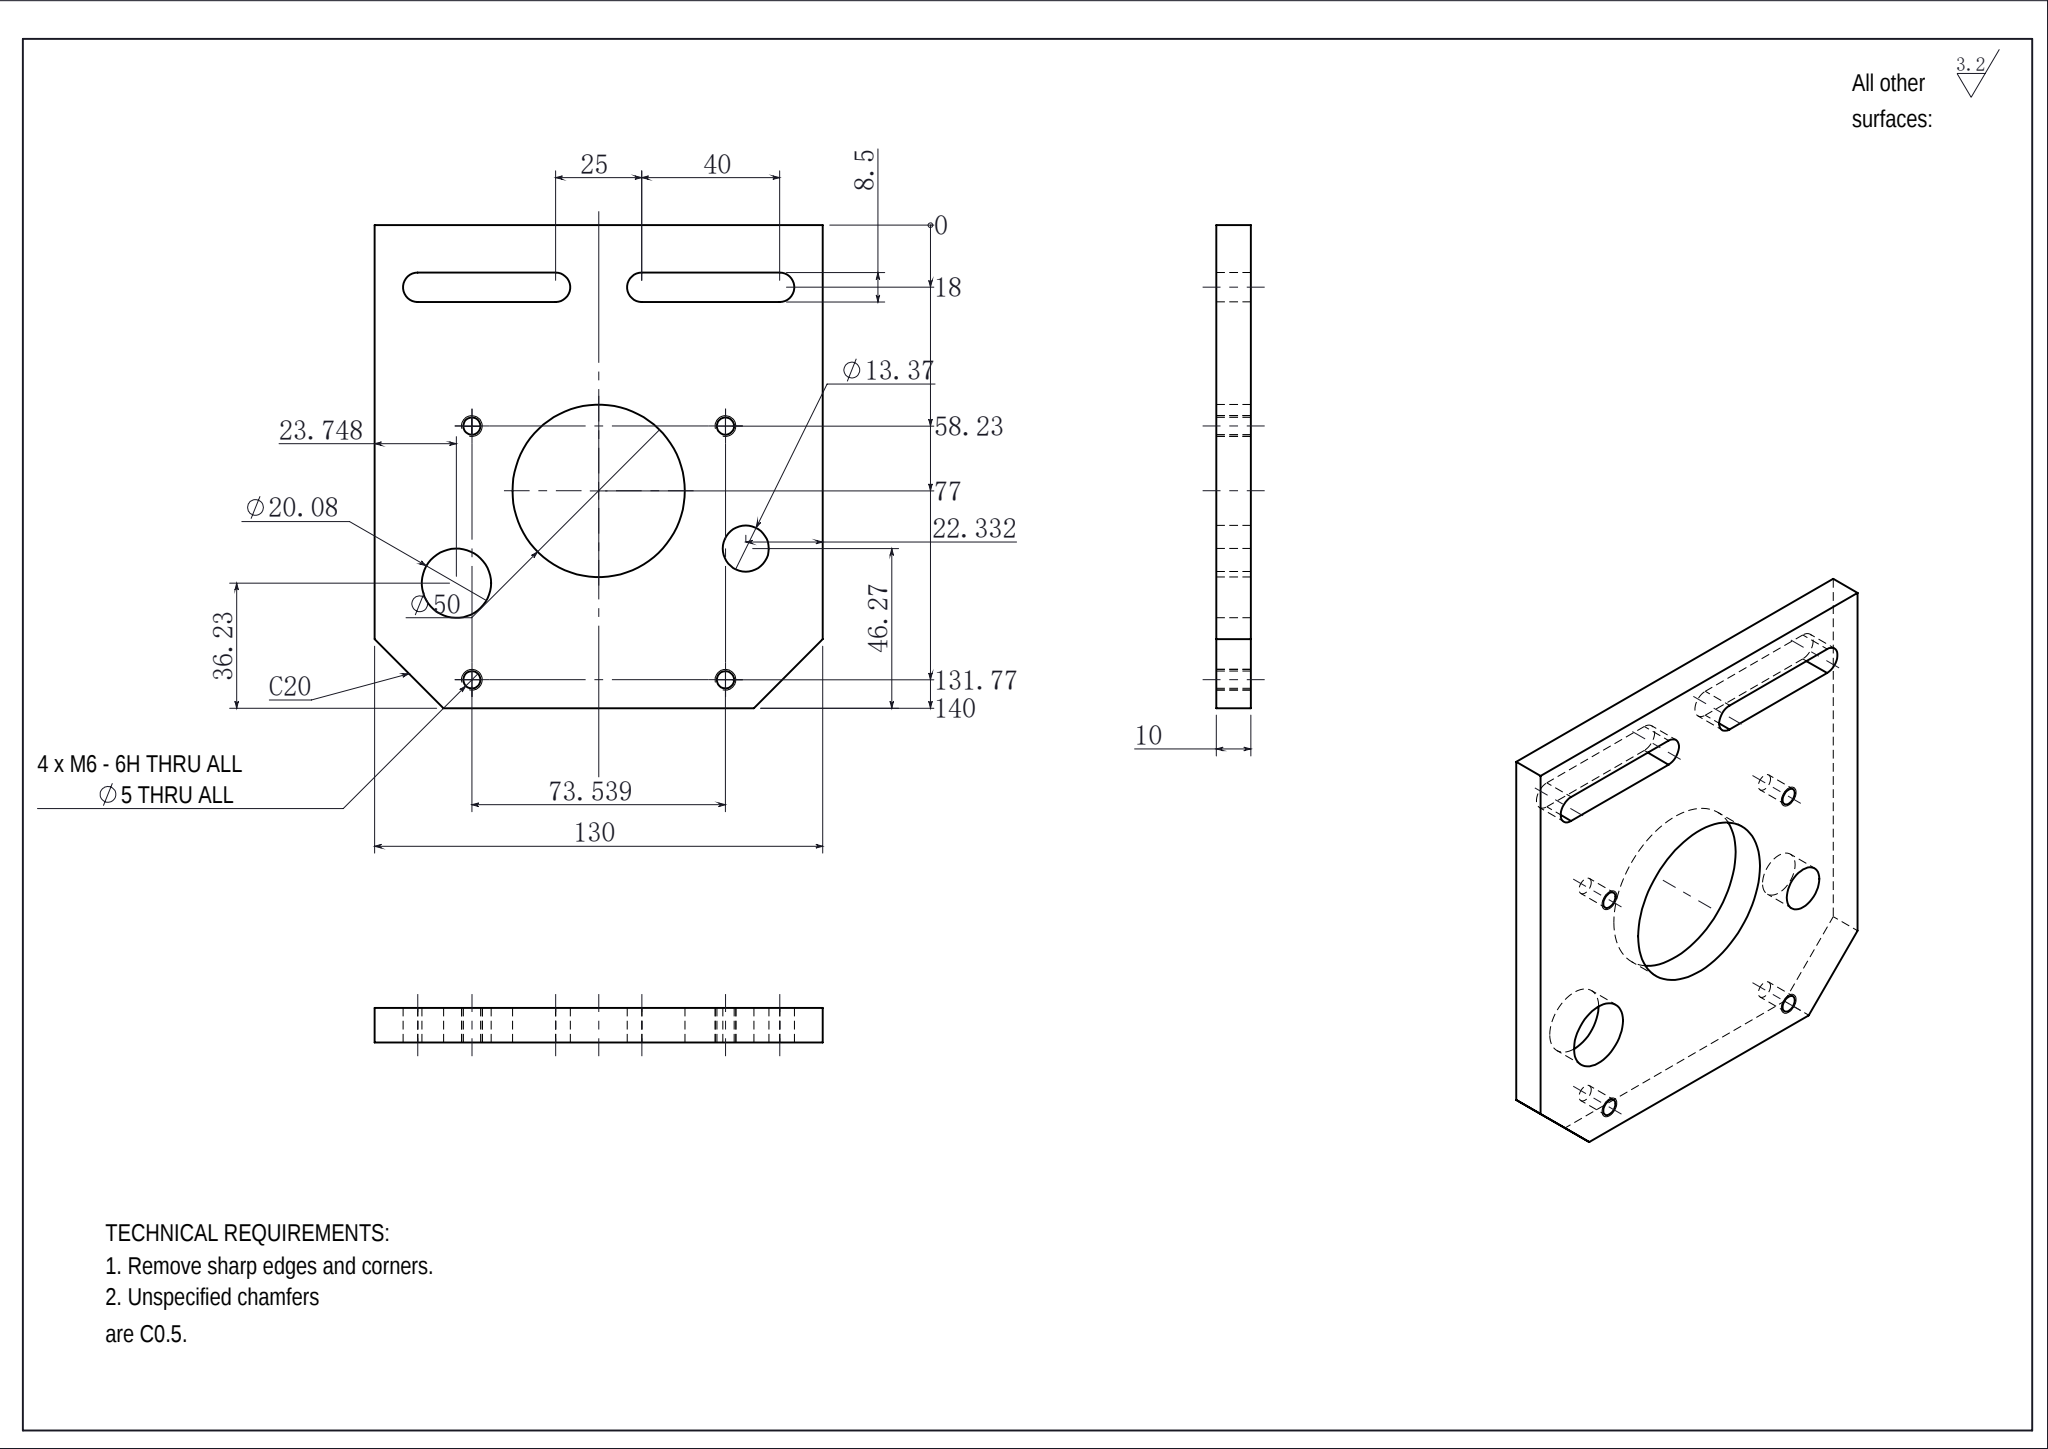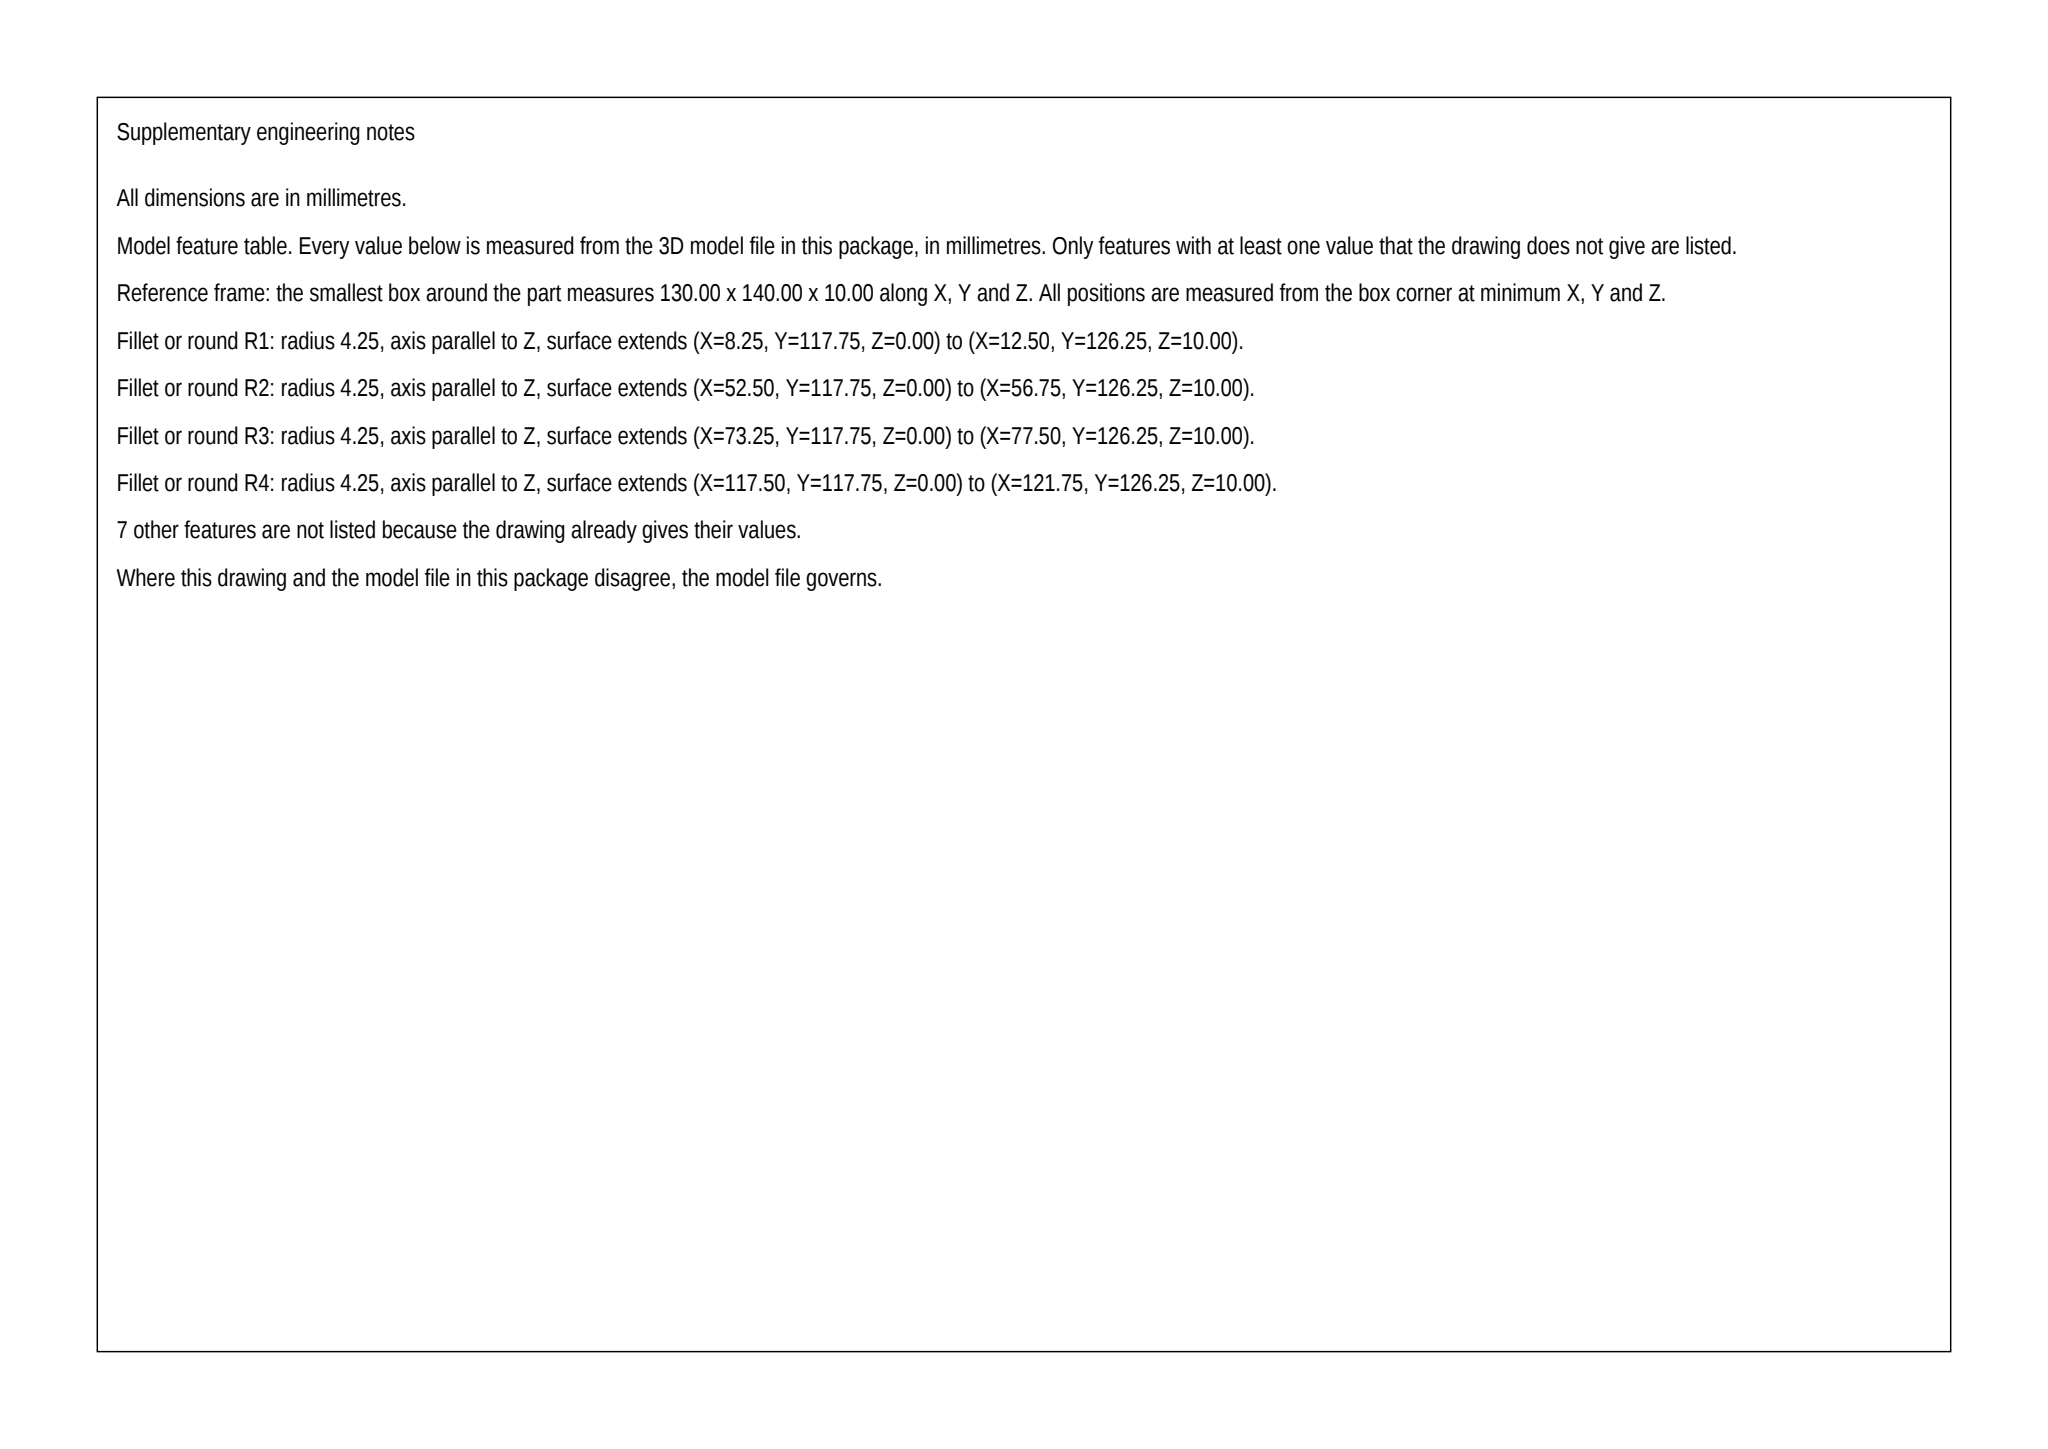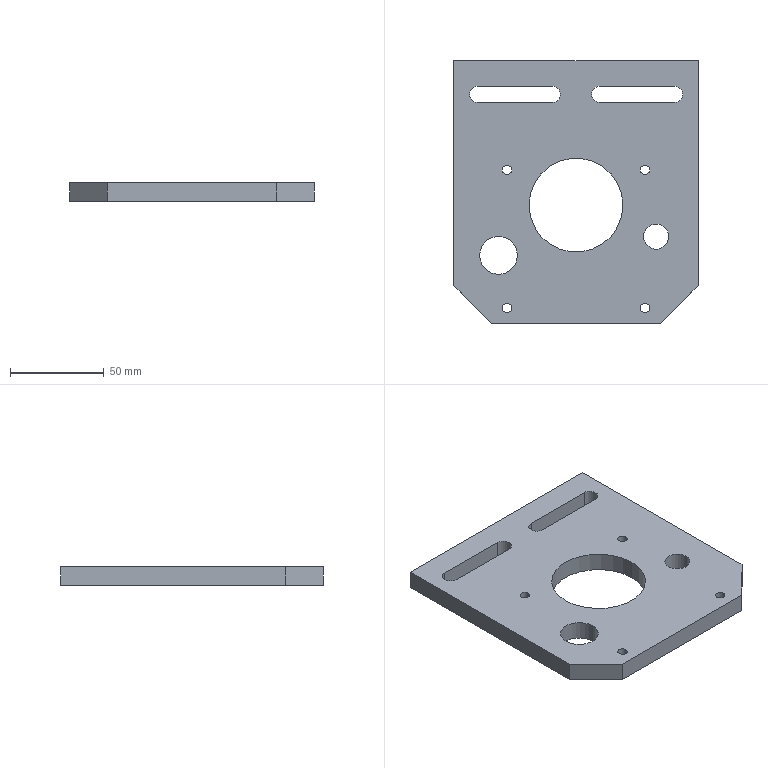Part | SolidWorks | mm | 1 solid | 32 faces | box 130 x 140 x 10 mm | volume 145074 mm3 | cylinder 20 | plane 12 | commonest cylinder face diameters 5 x8 8.5 x6 20.08 x2 13.37 x2 50 x2
build123d program:
from build123d import *

# Parameters (mm, degrees)
SKETCH1_W           = 130
SKETCH1_H           = 140
BOSS_EXTRUDE1_DEPTH = 5
CUT_EXTRUDE1_DEPTH  = 114
CHAMFER1_SIZE       = 20
M6_TAPPED_HOLE1_D   = 5
SKETCH9_R           = 25
CUT_EXTRUDE2_DEPTH  = 107
SKETCH10_R          = 10.04
SKETCH10_R_2        = 6.685
CUT_EXTRUDE3_DEPTH  = 80


with BuildPart() as part:
    # Sketch1 → Boss-Extrude1 (new, symmetric)
    with BuildSketch(Plane.XY):
        Rectangle(SKETCH1_W, SKETCH1_H)
    extrude(amount=BOSS_EXTRUDE1_DEPTH, both=True)

    # Sketch6 → Cut-Extrude1 (cut)
    with BuildSketch(Plane(origin=(0, 0, -5), x_dir=(-1, 0, 0), z_dir=(0, 0, -1))):
        with BuildLine():
            Line((-52.5, 56.25), (-12.5, 56.25))
            ThreePointArc((-12.5, 56.25), (-8.25, 52), (-12.5, 47.75))
            Line((-12.5, 47.75), (-52.5, 47.75))
            ThreePointArc((-52.5, 47.75), (-56.75, 52), (-52.5, 56.25))
        make_face()
        with BuildLine():
            Line((52.5, 56.25), (12.5, 56.25))
            ThreePointArc((12.5, 56.25), (8.25, 52), (12.5, 47.75))
            Line((12.5, 47.75), (52.5, 47.75))
            ThreePointArc((52.5, 47.75), (56.75, 52), (52.5, 56.25))
        make_face()
    extrude(amount=-CUT_EXTRUDE1_DEPTH, mode=Mode.SUBTRACT)

    # Chamfer1
    chamfer1_edges = [part.edges().sort_by_distance(p)[0] for p in [
        (65, -70, 0),
        (-65, -70, 0),
    ]]
    chamfer(chamfer1_edges, length=CHAMFER1_SIZE)

    # M6 Tapped Hole1 (through all)
    with Locations(Plane.XY.offset(5)):
        with Locations((36.77, 11.77), (-36.77, 11.77), (-36.77, -61.77), (36.77, -61.77)):
            Hole(M6_TAPPED_HOLE1_D / 2)

    # Sketch9 → Cut-Extrude2 (cut)
    with BuildSketch(Plane(origin=(0, 0, -5), x_dir=(-1, 0, 0), z_dir=(0, 0, -1))):
        with Locations((0, -7)):
            Circle(SKETCH9_R)
    extrude(amount=-CUT_EXTRUDE2_DEPTH, mode=Mode.SUBTRACT)

    # Sketch10 → Cut-Extrude3 (cut)
    with BuildSketch(Plane.XY.offset(5)):
        with Locations((-41.252, -33.77)):
            Circle(SKETCH10_R)
        with Locations((42.668, -23.73)):
            Circle(SKETCH10_R_2)
    extrude(amount=-CUT_EXTRUDE3_DEPTH, mode=Mode.SUBTRACT)


solid = part.part